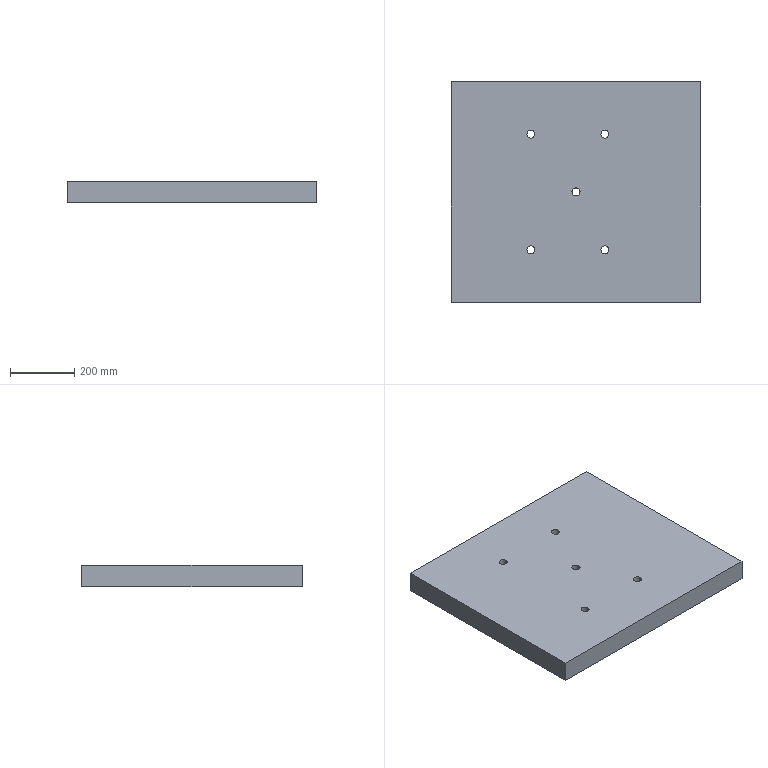Component | SolidWorks | Tray-1 | 1 solid | 16 faces | box 775 x 685 x 66 mm | volume 34875762 mm3 | cylinder 10 | plane 6 | commonest cylinder face diameters 25 x10
build123d program:
from build123d import *

# Parameters (mm, degrees)
SKETCH1_W                  = 775
SKETCH1_H                  = 685
BOSS_EXTRUDE1_DEPTH        = 66
F_25_0_25_DIAMETER_HOLE1_D = 25


with BuildPart() as part:
    # Sketch1 → Boss-Extrude1 (new body)
    with BuildSketch(Plane.XY):
        Rectangle(SKETCH1_W, SKETCH1_H)
    extrude(amount=BOSS_EXTRUDE1_DEPTH)

    # 25.0 _25_ Diameter Hole1 (through all)
    with Locations(Plane(origin=(0, 0, 0), x_dir=(-1, 0, 0), z_dir=(0, 0, -1))):
        with Locations((140, -180), (-90, -180), (-90, 180), (140, 180), (0, 0)):
            Hole(F_25_0_25_DIAMETER_HOLE1_D / 2)


solid = part.part

# Placed as in the assembly
solid = solid.moved(Location((44.708, 14.301, -492), (0, 0, 0)))
STEP:
#1=COLOUR_RGB('',0.7922,0.8196,0.9333);
#2=FILL_AREA_STYLE_COLOUR('',#1);
#3=FILL_AREA_STYLE('',(#2));
#4=SURFACE_STYLE_FILL_AREA(#3);
#5=SURFACE_SIDE_STYLE('',(#4));
#6=SURFACE_STYLE_USAGE(.BOTH.,#5);
#7=PRESENTATION_STYLE_ASSIGNMENT((#6));
#8=CARTESIAN_POINT('',(-3.26,-6.524,-16.772));
#9=VERTEX_POINT('',#8);
#10=CARTESIAN_POINT('',(-4.244,-6.524,-16.772));
#11=VERTEX_POINT('',#10);
#12=CARTESIAN_POINT('',(-3.752,-6.524,-16.772));
#13=DIRECTION('',(0.,0.,-1.));
#14=DIRECTION('',(-1.,0.,0.));
#15=AXIS2_PLACEMENT_3D('',#12,#13,#14);
#16=CIRCLE('',#15,0.4921);
#17=EDGE_CURVE('',#9,#11,#16,.T.);
#18=ORIENTED_EDGE('',*,*,#17,.F.);
#19=CARTESIAN_POINT('',(-3.26,-6.524,-19.37));
#20=VERTEX_POINT('',#19);
#21=CARTESIAN_POINT('',(-3.26,-6.524,-19.37));
#22=DIRECTION('',(0.,0.,-1.));
#23=VECTOR('',#22,39.37);
#24=LINE('',#21,#23);
#25=EDGE_CURVE('',#9,#20,#24,.T.);
#26=ORIENTED_EDGE('',*,*,#25,.T.);
#27=CARTESIAN_POINT('',(-4.244,-6.524,-19.37));
#28=VERTEX_POINT('',#27);
#29=CARTESIAN_POINT('',(-3.752,-6.524,-19.37));
#30=DIRECTION('',(0.,0.,-1.));
#31=DIRECTION('',(-1.,0.,0.));
#32=AXIS2_PLACEMENT_3D('',#29,#30,#31);
#33=CIRCLE('',#32,0.4921);
#34=EDGE_CURVE('',#20,#28,#33,.T.);
#35=ORIENTED_EDGE('',*,*,#34,.T.);
#36=CARTESIAN_POINT('',(-4.244,-6.524,-19.37));
#37=DIRECTION('',(0.,0.,-1.));
#38=VECTOR('',#37,39.37);
#39=LINE('',#36,#38);
#40=EDGE_CURVE('',#11,#28,#39,.T.);
#41=ORIENTED_EDGE('',*,*,#40,.F.);
#42=EDGE_LOOP('',(#18,#26,#35,#41));
#43=FACE_OUTER_BOUND('',#42,.T.);
#44=CARTESIAN_POINT('',(-3.752,-6.524,-19.37));
#45=DIRECTION('',(0.,0.,-1.));
#46=DIRECTION('',(-1.,0.,0.));
#47=AXIS2_PLACEMENT_3D('',#44,#45,#46);
#48=CYLINDRICAL_SURFACE('',#47,0.4921);
#49=ADVANCED_FACE('',(#43),#48,.F.);
#50=CARTESIAN_POINT('',(5.796,-6.524,-16.772));
#51=VERTEX_POINT('',#50);
#52=CARTESIAN_POINT('',(4.811,-6.524,-16.772));
#53=VERTEX_POINT('',#52);
#54=CARTESIAN_POINT('',(5.303,-6.524,-16.772));
#55=DIRECTION('',(0.,0.,-1.));
#56=DIRECTION('',(-1.,0.,0.));
#57=AXIS2_PLACEMENT_3D('',#54,#55,#56);
#58=CIRCLE('',#57,0.4921);
#59=EDGE_CURVE('',#51,#53,#58,.T.);
#60=ORIENTED_EDGE('',*,*,#59,.F.);
#61=CARTESIAN_POINT('',(5.796,-6.524,-19.37));
#62=VERTEX_POINT('',#61);
#63=CARTESIAN_POINT('',(5.796,-6.524,-19.37));
#64=DIRECTION('',(0.,0.,-1.));
#65=VECTOR('',#64,39.37);
#66=LINE('',#63,#65);
#67=EDGE_CURVE('',#51,#62,#66,.T.);
#68=ORIENTED_EDGE('',*,*,#67,.T.);
#69=CARTESIAN_POINT('',(4.811,-6.524,-19.37));
#70=VERTEX_POINT('',#69);
#71=CARTESIAN_POINT('',(5.303,-6.524,-19.37));
#72=DIRECTION('',(0.,0.,-1.));
#73=DIRECTION('',(-1.,0.,0.));
#74=AXIS2_PLACEMENT_3D('',#71,#72,#73);
#75=CIRCLE('',#74,0.4921);
#76=EDGE_CURVE('',#62,#70,#75,.T.);
#77=ORIENTED_EDGE('',*,*,#76,.T.);
#78=CARTESIAN_POINT('',(4.811,-6.524,-19.37));
#79=DIRECTION('',(0.,0.,-1.));
#80=VECTOR('',#79,39.37);
#81=LINE('',#78,#80);
#82=EDGE_CURVE('',#53,#70,#81,.T.);
#83=ORIENTED_EDGE('',*,*,#82,.F.);
#84=EDGE_LOOP('',(#60,#68,#77,#83));
#85=FACE_OUTER_BOUND('',#84,.T.);
#86=CARTESIAN_POINT('',(5.303,-6.524,-19.37));
#87=DIRECTION('',(0.,0.,-1.));
#88=DIRECTION('',(-1.,0.,0.));
#89=AXIS2_PLACEMENT_3D('',#86,#87,#88);
#90=CYLINDRICAL_SURFACE('',#89,0.4921);
#91=ADVANCED_FACE('',(#85),#90,.F.);
#92=CARTESIAN_POINT('',(5.796,7.65,-16.772));
#93=VERTEX_POINT('',#92);
#94=CARTESIAN_POINT('',(4.811,7.65,-16.772));
#95=VERTEX_POINT('',#94);
#96=CARTESIAN_POINT('',(5.303,7.65,-16.772));
#97=DIRECTION('',(0.,0.,-1.));
#98=DIRECTION('',(-1.,0.,0.));
#99=AXIS2_PLACEMENT_3D('',#96,#97,#98);
#100=CIRCLE('',#99,0.4921);
#101=EDGE_CURVE('',#93,#95,#100,.T.);
#102=ORIENTED_EDGE('',*,*,#101,.F.);
#103=CARTESIAN_POINT('',(5.796,7.65,-19.37));
#104=VERTEX_POINT('',#103);
#105=CARTESIAN_POINT('',(5.796,7.65,-19.37));
#106=DIRECTION('',(0.,0.,-1.));
#107=VECTOR('',#106,39.37);
#108=LINE('',#105,#107);
#109=EDGE_CURVE('',#93,#104,#108,.T.);
#110=ORIENTED_EDGE('',*,*,#109,.T.);
#111=CARTESIAN_POINT('',(4.811,7.65,-19.37));
#112=VERTEX_POINT('',#111);
#113=CARTESIAN_POINT('',(5.303,7.65,-19.37));
#114=DIRECTION('',(0.,0.,-1.));
#115=DIRECTION('',(-1.,0.,0.));
#116=AXIS2_PLACEMENT_3D('',#113,#114,#115);
#117=CIRCLE('',#116,0.4921);
#118=EDGE_CURVE('',#104,#112,#117,.T.);
#119=ORIENTED_EDGE('',*,*,#118,.T.);
#120=CARTESIAN_POINT('',(4.811,7.65,-19.37));
#121=DIRECTION('',(0.,0.,-1.));
#122=VECTOR('',#121,39.37);
#123=LINE('',#120,#122);
#124=EDGE_CURVE('',#95,#112,#123,.T.);
#125=ORIENTED_EDGE('',*,*,#124,.F.);
#126=EDGE_LOOP('',(#102,#110,#119,#125));
#127=FACE_OUTER_BOUND('',#126,.T.);
#128=CARTESIAN_POINT('',(5.303,7.65,-19.37));
#129=DIRECTION('',(0.,0.,-1.));
#130=DIRECTION('',(-1.,0.,0.));
#131=AXIS2_PLACEMENT_3D('',#128,#129,#130);
#132=CYLINDRICAL_SURFACE('',#131,0.4921);
#133=ADVANCED_FACE('',(#127),#132,.F.);
#134=CARTESIAN_POINT('',(-3.26,7.65,-16.772));
#135=VERTEX_POINT('',#134);
#136=CARTESIAN_POINT('',(-4.244,7.65,-16.772));
#137=VERTEX_POINT('',#136);
#138=CARTESIAN_POINT('',(-3.752,7.65,-16.772));
#139=DIRECTION('',(0.,0.,-1.));
#140=DIRECTION('',(-1.,0.,0.));
#141=AXIS2_PLACEMENT_3D('',#138,#139,#140);
#142=CIRCLE('',#141,0.4921);
#143=EDGE_CURVE('',#135,#137,#142,.T.);
#144=ORIENTED_EDGE('',*,*,#143,.F.);
#145=CARTESIAN_POINT('',(-3.26,7.65,-19.37));
#146=VERTEX_POINT('',#145);
#147=CARTESIAN_POINT('',(-3.26,7.65,-19.37));
#148=DIRECTION('',(0.,0.,-1.));
#149=VECTOR('',#148,39.37);
#150=LINE('',#147,#149);
#151=EDGE_CURVE('',#135,#146,#150,.T.);
#152=ORIENTED_EDGE('',*,*,#151,.T.);
#153=CARTESIAN_POINT('',(-4.244,7.65,-19.37));
#154=VERTEX_POINT('',#153);
#155=CARTESIAN_POINT('',(-3.752,7.65,-19.37));
#156=DIRECTION('',(0.,0.,-1.));
#157=DIRECTION('',(-1.,0.,0.));
#158=AXIS2_PLACEMENT_3D('',#155,#156,#157);
#159=CIRCLE('',#158,0.4921);
#160=EDGE_CURVE('',#146,#154,#159,.T.);
#161=ORIENTED_EDGE('',*,*,#160,.T.);
#162=CARTESIAN_POINT('',(-4.244,7.65,-19.37));
#163=DIRECTION('',(0.,0.,-1.));
#164=VECTOR('',#163,39.37);
#165=LINE('',#162,#164);
#166=EDGE_CURVE('',#137,#154,#165,.T.);
#167=ORIENTED_EDGE('',*,*,#166,.F.);
#168=EDGE_LOOP('',(#144,#152,#161,#167));
#169=FACE_OUTER_BOUND('',#168,.T.);
#170=CARTESIAN_POINT('',(-3.752,7.65,-19.37));
#171=DIRECTION('',(0.,0.,-1.));
#172=DIRECTION('',(-1.,0.,0.));
#173=AXIS2_PLACEMENT_3D('',#170,#171,#172);
#174=CYLINDRICAL_SURFACE('',#173,0.4921);
#175=ADVANCED_FACE('',(#169),#174,.F.);
#176=CARTESIAN_POINT('',(2.252,0.563,-16.772));
#177=VERTEX_POINT('',#176);
#178=CARTESIAN_POINT('',(1.268,0.563,-16.772));
#179=VERTEX_POINT('',#178);
#180=CARTESIAN_POINT('',(1.76,0.563,-16.772));
#181=DIRECTION('',(0.,0.,-1.));
#182=DIRECTION('',(-1.,0.,0.));
#183=AXIS2_PLACEMENT_3D('',#180,#181,#182);
#184=CIRCLE('',#183,0.4921);
#185=EDGE_CURVE('',#177,#179,#184,.T.);
#186=ORIENTED_EDGE('',*,*,#185,.F.);
#187=CARTESIAN_POINT('',(2.252,0.563,-19.37));
#188=VERTEX_POINT('',#187);
#189=CARTESIAN_POINT('',(2.252,0.563,-19.37));
#190=DIRECTION('',(0.,0.,-1.));
#191=VECTOR('',#190,39.37);
#192=LINE('',#189,#191);
#193=EDGE_CURVE('',#177,#188,#192,.T.);
#194=ORIENTED_EDGE('',*,*,#193,.T.);
#195=CARTESIAN_POINT('',(1.268,0.563,-19.37));
#196=VERTEX_POINT('',#195);
#197=CARTESIAN_POINT('',(1.76,0.563,-19.37));
#198=DIRECTION('',(0.,0.,-1.));
#199=DIRECTION('',(-1.,0.,0.));
#200=AXIS2_PLACEMENT_3D('',#197,#198,#199);
#201=CIRCLE('',#200,0.4921);
#202=EDGE_CURVE('',#188,#196,#201,.T.);
#203=ORIENTED_EDGE('',*,*,#202,.T.);
#204=CARTESIAN_POINT('',(1.268,0.563,-19.37));
#205=DIRECTION('',(0.,0.,-1.));
#206=VECTOR('',#205,39.37);
#207=LINE('',#204,#206);
#208=EDGE_CURVE('',#179,#196,#207,.T.);
#209=ORIENTED_EDGE('',*,*,#208,.F.);
#210=EDGE_LOOP('',(#186,#194,#203,#209));
#211=FACE_OUTER_BOUND('',#210,.T.);
#212=CARTESIAN_POINT('',(1.76,0.563,-19.37));
#213=DIRECTION('',(0.,0.,-1.));
#214=DIRECTION('',(-1.,0.,0.));
#215=AXIS2_PLACEMENT_3D('',#212,#213,#214);
#216=CYLINDRICAL_SURFACE('',#215,0.4921);
#217=ADVANCED_FACE('',(#211),#216,.F.);
#218=CARTESIAN_POINT('',(-3.752,-6.524,-19.37));
#219=DIRECTION('',(0.,0.,-1.));
#220=DIRECTION('',(-1.,0.,0.));
#221=AXIS2_PLACEMENT_3D('',#218,#219,#220);
#222=CIRCLE('',#221,0.4921);
#223=EDGE_CURVE('',#28,#20,#222,.T.);
#224=ORIENTED_EDGE('',*,*,#223,.F.);
#225=ORIENTED_EDGE('',*,*,#34,.F.);
#226=EDGE_LOOP('',(#224,#225));
#227=FACE_BOUND('',#226,.T.);
#228=CARTESIAN_POINT('',(5.303,-6.524,-19.37));
#229=DIRECTION('',(0.,0.,-1.));
#230=DIRECTION('',(-1.,0.,0.));
#231=AXIS2_PLACEMENT_3D('',#228,#229,#230);
#232=CIRCLE('',#231,0.4921);
#233=EDGE_CURVE('',#70,#62,#232,.T.);
#234=ORIENTED_EDGE('',*,*,#233,.F.);
#235=ORIENTED_EDGE('',*,*,#76,.F.);
#236=EDGE_LOOP('',(#234,#235));
#237=FACE_BOUND('',#236,.T.);
#238=CARTESIAN_POINT('',(5.303,7.65,-19.37));
#239=DIRECTION('',(0.,0.,-1.));
#240=DIRECTION('',(-1.,0.,0.));
#241=AXIS2_PLACEMENT_3D('',#238,#239,#240);
#242=CIRCLE('',#241,0.4921);
#243=EDGE_CURVE('',#112,#104,#242,.T.);
#244=ORIENTED_EDGE('',*,*,#243,.F.);
#245=ORIENTED_EDGE('',*,*,#118,.F.);
#246=EDGE_LOOP('',(#244,#245));
#247=FACE_BOUND('',#246,.T.);
#248=CARTESIAN_POINT('',(-3.752,7.65,-19.37));
#249=DIRECTION('',(0.,0.,-1.));
#250=DIRECTION('',(-1.,0.,0.));
#251=AXIS2_PLACEMENT_3D('',#248,#249,#250);
#252=CIRCLE('',#251,0.4921);
#253=EDGE_CURVE('',#154,#146,#252,.T.);
#254=ORIENTED_EDGE('',*,*,#253,.F.);
#255=ORIENTED_EDGE('',*,*,#160,.F.);
#256=EDGE_LOOP('',(#254,#255));
#257=FACE_BOUND('',#256,.T.);
#258=CARTESIAN_POINT('',(-13.496,14.047,-19.37));
#259=VERTEX_POINT('',#258);
#260=CARTESIAN_POINT('',(-13.496,-12.921,-19.37));
#261=VERTEX_POINT('',#260);
#262=CARTESIAN_POINT('',(-13.496,-12.921,-19.37));
#263=DIRECTION('',(0.,-1.,0.));
#264=VECTOR('',#263,39.37);
#265=LINE('',#262,#264);
#266=EDGE_CURVE('',#259,#261,#265,.T.);
#267=ORIENTED_EDGE('',*,*,#266,.F.);
#268=CARTESIAN_POINT('',(17.016,14.047,-19.37));
#269=VERTEX_POINT('',#268);
#270=CARTESIAN_POINT('',(17.016,14.047,-19.37));
#271=DIRECTION('',(-1.,-0.,0.));
#272=VECTOR('',#271,39.37);
#273=LINE('',#270,#272);
#274=EDGE_CURVE('',#269,#259,#273,.T.);
#275=ORIENTED_EDGE('',*,*,#274,.F.);
#276=CARTESIAN_POINT('',(17.016,-12.921,-19.37));
#277=VERTEX_POINT('',#276);
#278=CARTESIAN_POINT('',(17.016,-12.921,-19.37));
#279=DIRECTION('',(0.,1.,0.));
#280=VECTOR('',#279,39.37);
#281=LINE('',#278,#280);
#282=EDGE_CURVE('',#277,#269,#281,.T.);
#283=ORIENTED_EDGE('',*,*,#282,.F.);
#284=CARTESIAN_POINT('',(17.016,-12.921,-19.37));
#285=DIRECTION('',(1.,0.,0.));
#286=VECTOR('',#285,39.37);
#287=LINE('',#284,#286);
#288=EDGE_CURVE('',#261,#277,#287,.T.);
#289=ORIENTED_EDGE('',*,*,#288,.F.);
#290=EDGE_LOOP('',(#267,#275,#283,#289));
#291=FACE_OUTER_BOUND('',#290,.T.);
#292=CARTESIAN_POINT('',(1.76,0.563,-19.37));
#293=DIRECTION('',(0.,0.,-1.));
#294=DIRECTION('',(-1.,0.,0.));
#295=AXIS2_PLACEMENT_3D('',#292,#293,#294);
#296=CIRCLE('',#295,0.4921);
#297=EDGE_CURVE('',#196,#188,#296,.T.);
#298=ORIENTED_EDGE('',*,*,#297,.F.);
#299=ORIENTED_EDGE('',*,*,#202,.F.);
#300=EDGE_LOOP('',(#298,#299));
#301=FACE_BOUND('',#300,.T.);
#302=CARTESIAN_POINT('',(1.76,0.563,-19.37));
#303=DIRECTION('',(0.,0.,1.));
#304=DIRECTION('',(1.,0.,0.));
#305=AXIS2_PLACEMENT_3D('',#302,#303,#304);
#306=PLANE('',#305);
#307=ADVANCED_FACE('',(#227,#237,#247,#257,#291,#301),#306,.F.);
#308=ORIENTED_EDGE('',*,*,#266,.T.);
#309=CARTESIAN_POINT('',(-13.496,-12.921,-16.772));
#310=VERTEX_POINT('',#309);
#311=CARTESIAN_POINT('',(-13.496,-12.921,-16.772));
#312=DIRECTION('',(0.,0.,-1.));
#313=VECTOR('',#312,39.37);
#314=LINE('',#311,#313);
#315=EDGE_CURVE('',#310,#261,#314,.T.);
#316=ORIENTED_EDGE('',*,*,#315,.F.);
#317=CARTESIAN_POINT('',(-13.496,14.047,-16.772));
#318=VERTEX_POINT('',#317);
#319=CARTESIAN_POINT('',(-13.496,-12.921,-16.772));
#320=DIRECTION('',(0.,-1.,0.));
#321=VECTOR('',#320,39.37);
#322=LINE('',#319,#321);
#323=EDGE_CURVE('',#318,#310,#322,.T.);
#324=ORIENTED_EDGE('',*,*,#323,.F.);
#325=CARTESIAN_POINT('',(-13.496,14.047,-16.772));
#326=DIRECTION('',(0.,0.,-1.));
#327=VECTOR('',#326,39.37);
#328=LINE('',#325,#327);
#329=EDGE_CURVE('',#318,#259,#328,.T.);
#330=ORIENTED_EDGE('',*,*,#329,.T.);
#331=EDGE_LOOP('',(#308,#316,#324,#330));
#332=FACE_OUTER_BOUND('',#331,.T.);
#333=CARTESIAN_POINT('',(-13.496,-12.921,-16.772));
#334=DIRECTION('',(1.,0.,0.));
#335=DIRECTION('',(0.,0.,-1.));
#336=AXIS2_PLACEMENT_3D('',#333,#334,#335);
#337=PLANE('',#336);
#338=ADVANCED_FACE('',(#332),#337,.F.);
#339=ORIENTED_EDGE('',*,*,#288,.T.);
#340=CARTESIAN_POINT('',(17.016,-12.921,-16.772));
#341=VERTEX_POINT('',#340);
#342=CARTESIAN_POINT('',(17.016,-12.921,-16.772));
#343=DIRECTION('',(0.,0.,-1.));
#344=VECTOR('',#343,39.37);
#345=LINE('',#342,#344);
#346=EDGE_CURVE('',#341,#277,#345,.T.);
#347=ORIENTED_EDGE('',*,*,#346,.F.);
#348=CARTESIAN_POINT('',(17.016,-12.921,-16.772));
#349=DIRECTION('',(1.,0.,0.));
#350=VECTOR('',#349,39.37);
#351=LINE('',#348,#350);
#352=EDGE_CURVE('',#310,#341,#351,.T.);
#353=ORIENTED_EDGE('',*,*,#352,.F.);
#354=ORIENTED_EDGE('',*,*,#315,.T.);
#355=EDGE_LOOP('',(#339,#347,#353,#354));
#356=FACE_OUTER_BOUND('',#355,.T.);
#357=CARTESIAN_POINT('',(17.016,-12.921,-16.772));
#358=DIRECTION('',(-0.,1.,0.));
#359=DIRECTION('',(-1.,-0.,0.));
#360=AXIS2_PLACEMENT_3D('',#357,#358,#359);
#361=PLANE('',#360);
#362=ADVANCED_FACE('',(#356),#361,.F.);
#363=ORIENTED_EDGE('',*,*,#282,.T.);
#364=CARTESIAN_POINT('',(17.016,14.047,-16.772));
#365=VERTEX_POINT('',#364);
#366=CARTESIAN_POINT('',(17.016,14.047,-16.772));
#367=DIRECTION('',(0.,0.,-1.));
#368=VECTOR('',#367,39.37);
#369=LINE('',#366,#368);
#370=EDGE_CURVE('',#365,#269,#369,.T.);
#371=ORIENTED_EDGE('',*,*,#370,.F.);
#372=CARTESIAN_POINT('',(17.016,-12.921,-16.772));
#373=DIRECTION('',(0.,1.,0.));
#374=VECTOR('',#373,39.37);
#375=LINE('',#372,#374);
#376=EDGE_CURVE('',#341,#365,#375,.T.);
#377=ORIENTED_EDGE('',*,*,#376,.F.);
#378=ORIENTED_EDGE('',*,*,#346,.T.);
#379=EDGE_LOOP('',(#363,#371,#377,#378));
#380=FACE_OUTER_BOUND('',#379,.T.);
#381=CARTESIAN_POINT('',(17.016,-12.921,-16.772));
#382=DIRECTION('',(-1.,0.,0.));
#383=DIRECTION('',(0.,0.,1.));
#384=AXIS2_PLACEMENT_3D('',#381,#382,#383);
#385=PLANE('',#384);
#386=ADVANCED_FACE('',(#380),#385,.F.);
#387=ORIENTED_EDGE('',*,*,#274,.T.);
#388=ORIENTED_EDGE('',*,*,#329,.F.);
#389=CARTESIAN_POINT('',(17.016,14.047,-16.772));
#390=DIRECTION('',(-1.,-0.,0.));
#391=VECTOR('',#390,39.37);
#392=LINE('',#389,#391);
#393=EDGE_CURVE('',#365,#318,#392,.T.);
#394=ORIENTED_EDGE('',*,*,#393,.F.);
#395=ORIENTED_EDGE('',*,*,#370,.T.);
#396=EDGE_LOOP('',(#387,#388,#394,#395));
#397=FACE_OUTER_BOUND('',#396,.T.);
#398=CARTESIAN_POINT('',(17.016,14.047,-16.772));
#399=DIRECTION('',(0.,-1.,0.));
#400=DIRECTION('',(1.,0.,0.));
#401=AXIS2_PLACEMENT_3D('',#398,#399,#400);
#402=PLANE('',#401);
#403=ADVANCED_FACE('',(#397),#402,.F.);
#404=CARTESIAN_POINT('',(-3.752,-6.524,-16.772));
#405=DIRECTION('',(0.,0.,-1.));
#406=DIRECTION('',(-1.,0.,0.));
#407=AXIS2_PLACEMENT_3D('',#404,#405,#406);
#408=CIRCLE('',#407,0.4921);
#409=EDGE_CURVE('',#11,#9,#408,.T.);
#410=ORIENTED_EDGE('',*,*,#409,.T.);
#411=ORIENTED_EDGE('',*,*,#17,.T.);
#412=EDGE_LOOP('',(#410,#411));
#413=FACE_BOUND('',#412,.T.);
#414=CARTESIAN_POINT('',(5.303,-6.524,-16.772));
#415=DIRECTION('',(0.,0.,-1.));
#416=DIRECTION('',(-1.,0.,0.));
#417=AXIS2_PLACEMENT_3D('',#414,#415,#416);
#418=CIRCLE('',#417,0.4921);
#419=EDGE_CURVE('',#53,#51,#418,.T.);
#420=ORIENTED_EDGE('',*,*,#419,.T.);
#421=ORIENTED_EDGE('',*,*,#59,.T.);
#422=EDGE_LOOP('',(#420,#421));
#423=FACE_BOUND('',#422,.T.);
#424=CARTESIAN_POINT('',(5.303,7.65,-16.772));
#425=DIRECTION('',(0.,0.,-1.));
#426=DIRECTION('',(-1.,0.,0.));
#427=AXIS2_PLACEMENT_3D('',#424,#425,#426);
#428=CIRCLE('',#427,0.4921);
#429=EDGE_CURVE('',#95,#93,#428,.T.);
#430=ORIENTED_EDGE('',*,*,#429,.T.);
#431=ORIENTED_EDGE('',*,*,#101,.T.);
#432=EDGE_LOOP('',(#430,#431));
#433=FACE_BOUND('',#432,.T.);
#434=CARTESIAN_POINT('',(-3.752,7.65,-16.772));
#435=DIRECTION('',(0.,0.,-1.));
#436=DIRECTION('',(-1.,0.,0.));
#437=AXIS2_PLACEMENT_3D('',#434,#435,#436);
#438=CIRCLE('',#437,0.4921);
#439=EDGE_CURVE('',#137,#135,#438,.T.);
#440=ORIENTED_EDGE('',*,*,#439,.T.);
#441=ORIENTED_EDGE('',*,*,#143,.T.);
#442=EDGE_LOOP('',(#440,#441));
#443=FACE_BOUND('',#442,.T.);
#444=CARTESIAN_POINT('',(1.76,0.563,-16.772));
#445=DIRECTION('',(0.,0.,-1.));
#446=DIRECTION('',(-1.,0.,0.));
#447=AXIS2_PLACEMENT_3D('',#444,#445,#446);
#448=CIRCLE('',#447,0.4921);
#449=EDGE_CURVE('',#179,#177,#448,.T.);
#450=ORIENTED_EDGE('',*,*,#449,.T.);
#451=ORIENTED_EDGE('',*,*,#185,.T.);
#452=EDGE_LOOP('',(#450,#451));
#453=FACE_BOUND('',#452,.T.);
#454=ORIENTED_EDGE('',*,*,#323,.T.);
#455=ORIENTED_EDGE('',*,*,#352,.T.);
#456=ORIENTED_EDGE('',*,*,#376,.T.);
#457=ORIENTED_EDGE('',*,*,#393,.T.);
#458=EDGE_LOOP('',(#454,#455,#456,#457));
#459=FACE_OUTER_BOUND('',#458,.T.);
#460=CARTESIAN_POINT('',(1.76,0.563,-16.772));
#461=DIRECTION('',(0.,0.,1.));
#462=DIRECTION('',(1.,0.,0.));
#463=AXIS2_PLACEMENT_3D('',#460,#461,#462);
#464=PLANE('',#463);
#465=ADVANCED_FACE('',(#413,#423,#433,#443,#453,#459),#464,.T.);
#466=ORIENTED_EDGE('',*,*,#193,.F.);
#467=ORIENTED_EDGE('',*,*,#449,.F.);
#468=ORIENTED_EDGE('',*,*,#208,.T.);
#469=ORIENTED_EDGE('',*,*,#297,.T.);
#470=EDGE_LOOP('',(#466,#467,#468,#469));
#471=FACE_OUTER_BOUND('',#470,.T.);
#472=CARTESIAN_POINT('',(1.76,0.563,-19.37));
#473=DIRECTION('',(0.,0.,-1.));
#474=DIRECTION('',(-1.,0.,0.));
#475=AXIS2_PLACEMENT_3D('',#472,#473,#474);
#476=CYLINDRICAL_SURFACE('',#475,0.4921);
#477=ADVANCED_FACE('',(#471),#476,.F.);
#478=ORIENTED_EDGE('',*,*,#151,.F.);
#479=ORIENTED_EDGE('',*,*,#439,.F.);
#480=ORIENTED_EDGE('',*,*,#166,.T.);
#481=ORIENTED_EDGE('',*,*,#253,.T.);
#482=EDGE_LOOP('',(#478,#479,#480,#481));
#483=FACE_OUTER_BOUND('',#482,.T.);
#484=CARTESIAN_POINT('',(-3.752,7.65,-19.37));
#485=DIRECTION('',(0.,0.,-1.));
#486=DIRECTION('',(-1.,0.,0.));
#487=AXIS2_PLACEMENT_3D('',#484,#485,#486);
#488=CYLINDRICAL_SURFACE('',#487,0.4921);
#489=ADVANCED_FACE('',(#483),#488,.F.);
#490=ORIENTED_EDGE('',*,*,#109,.F.);
#491=ORIENTED_EDGE('',*,*,#429,.F.);
#492=ORIENTED_EDGE('',*,*,#124,.T.);
#493=ORIENTED_EDGE('',*,*,#243,.T.);
#494=EDGE_LOOP('',(#490,#491,#492,#493));
#495=FACE_OUTER_BOUND('',#494,.T.);
#496=CARTESIAN_POINT('',(5.303,7.65,-19.37));
#497=DIRECTION('',(0.,0.,-1.));
#498=DIRECTION('',(-1.,0.,0.));
#499=AXIS2_PLACEMENT_3D('',#496,#497,#498);
#500=CYLINDRICAL_SURFACE('',#499,0.4921);
#501=ADVANCED_FACE('',(#495),#500,.F.);
#502=ORIENTED_EDGE('',*,*,#67,.F.);
#503=ORIENTED_EDGE('',*,*,#419,.F.);
#504=ORIENTED_EDGE('',*,*,#82,.T.);
#505=ORIENTED_EDGE('',*,*,#233,.T.);
#506=EDGE_LOOP('',(#502,#503,#504,#505));
#507=FACE_OUTER_BOUND('',#506,.T.);
#508=CARTESIAN_POINT('',(5.303,-6.524,-19.37));
#509=DIRECTION('',(0.,0.,-1.));
#510=DIRECTION('',(-1.,0.,0.));
#511=AXIS2_PLACEMENT_3D('',#508,#509,#510);
#512=CYLINDRICAL_SURFACE('',#511,0.4921);
#513=ADVANCED_FACE('',(#507),#512,.F.);
#514=ORIENTED_EDGE('',*,*,#25,.F.);
#515=ORIENTED_EDGE('',*,*,#409,.F.);
#516=ORIENTED_EDGE('',*,*,#40,.T.);
#517=ORIENTED_EDGE('',*,*,#223,.T.);
#518=EDGE_LOOP('',(#514,#515,#516,#517));
#519=FACE_OUTER_BOUND('',#518,.T.);
#520=CARTESIAN_POINT('',(-3.752,-6.524,-19.37));
#521=DIRECTION('',(0.,0.,-1.));
#522=DIRECTION('',(-1.,0.,0.));
#523=AXIS2_PLACEMENT_3D('',#520,#521,#522);
#524=CYLINDRICAL_SURFACE('',#523,0.4921);
#525=ADVANCED_FACE('',(#519),#524,.F.);
#526=CLOSED_SHELL('',(#49,#91,#133,#175,#217,#307,#338,#362,#386,#403,#465,#477,#489,#501,#513,#525));
#527=MANIFOLD_SOLID_BREP('',#526);
#528=STYLED_ITEM('',(#7),#527);
#529=PRESENTATION_LAYER_ASSIGNMENT('','',(#528));
#530=CARTESIAN_POINT('',(0.,0.,0.));
#531=DIRECTION('',(0.,0.,1.));
#532=DIRECTION('',(1.,0.,0.));
#533=AXIS2_PLACEMENT_3D('',#530,#531,#532);
#534=(LENGTH_UNIT()NAMED_UNIT(*)SI_UNIT($,.METRE.));
#535=LENGTH_MEASURE_WITH_UNIT(LENGTH_MEASURE(0.0254),#534);
#536=DIMENSIONAL_EXPONENTS(1.,0.,0.,0.,0.,0.,0.);
#537=(CONVERSION_BASED_UNIT('',#535)LENGTH_UNIT()NAMED_UNIT(#536));
#538=UNCERTAINTY_MEASURE_WITH_UNIT(LENGTH_MEASURE(0.00001),#537,'','');
#539=(NAMED_UNIT(*)PLANE_ANGLE_UNIT()SI_UNIT($,.RADIAN.));
#540=(NAMED_UNIT(*)SI_UNIT($,.STERADIAN.)SOLID_ANGLE_UNIT());
#541=(GEOMETRIC_REPRESENTATION_CONTEXT(3)GLOBAL_UNCERTAINTY_ASSIGNED_CONTEXT((#538))GLOBAL_UNIT_ASSIGNED_CONTEXT((#537,#539,#540))REPRESENTATION_CONTEXT('',''));
#542=ADVANCED_BREP_SHAPE_REPRESENTATION('',(#527,#533),#541);
#543=(LENGTH_UNIT()NAMED_UNIT(*)SI_UNIT($,.METRE.));
#544=LENGTH_MEASURE_WITH_UNIT(LENGTH_MEASURE(0.0254),#543);
#545=DIMENSIONAL_EXPONENTS(1.,0.,0.,0.,0.,0.,0.);
#546=(CONVERSION_BASED_UNIT('',#544)LENGTH_UNIT()NAMED_UNIT(#545));
#547=UNCERTAINTY_MEASURE_WITH_UNIT(LENGTH_MEASURE(0.00001),#546,'','');
#548=(NAMED_UNIT(*)PLANE_ANGLE_UNIT()SI_UNIT($,.RADIAN.));
#549=(NAMED_UNIT(*)SI_UNIT($,.STERADIAN.)SOLID_ANGLE_UNIT());
#550=(GEOMETRIC_REPRESENTATION_CONTEXT(3)GLOBAL_UNCERTAINTY_ASSIGNED_CONTEXT((#547))GLOBAL_UNIT_ASSIGNED_CONTEXT((#546,#548,#549))REPRESENTATION_CONTEXT('',''));
#551=MECHANICAL_DESIGN_GEOMETRIC_PRESENTATION_REPRESENTATION('',(#528),#550);